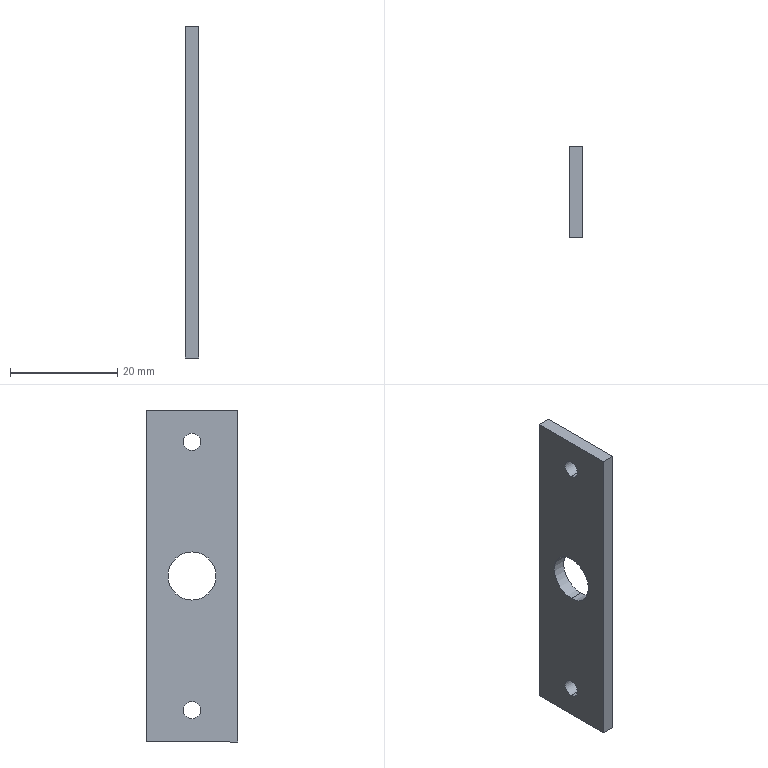Component | SolidWorks | BufferReinforcementPlate(PG50-106)-1 | 1 solid | 12 faces | box 2.5 x 17 x 61.9 mm | volume 2431 mm3 | cylinder 6 | plane 6 | commonest cylinder face diameters 3.2 x4 9 x2
build123d program:
from build123d import *

# Parameters (mm, degrees)
SKETCH1_W           = 61.9
SKETCH1_H           = 17
SKETCH1_R           = 1.6
SKETCH1_R_2         = 4.5
BOSS_EXTRUDE1_DEPTH = 2.5


with BuildPart() as part:
    # Sketch1 → Boss-Extrude1 (new body)
    with BuildSketch(Plane.XY):
        Rectangle(SKETCH1_W, SKETCH1_H)
        with Locations((-25, 0)):
            Circle(SKETCH1_R, mode=Mode.SUBTRACT)
        with Locations((25, 0)):
            Circle(SKETCH1_R, mode=Mode.SUBTRACT)
        Circle(SKETCH1_R_2, mode=Mode.SUBTRACT)
    extrude(amount=BOSS_EXTRUDE1_DEPTH)


solid = part.part

# Placed as in the assembly
solid = solid.moved(Location((919.318, -246.799, -300), (0, 90, 0)))
STEP:
#1=COLOUR_RGB('',0.7922,0.8196,0.9333);
#2=FILL_AREA_STYLE_COLOUR('',#1);
#3=FILL_AREA_STYLE('',(#2));
#4=SURFACE_STYLE_FILL_AREA(#3);
#5=SURFACE_SIDE_STYLE('',(#4));
#6=SURFACE_STYLE_USAGE(.BOTH.,#5);
#7=PRESENTATION_STYLE_ASSIGNMENT((#6));
#8=CARTESIAN_POINT('',(36.194,-9.716,-11.988));
#9=VERTEX_POINT('',#8);
#10=CARTESIAN_POINT('',(36.194,-9.716,-11.634));
#11=VERTEX_POINT('',#10);
#12=CARTESIAN_POINT('',(36.194,-9.716,-11.811));
#13=DIRECTION('',(-1.,0.,-0.));
#14=DIRECTION('',(0.,-0.,1.));
#15=AXIS2_PLACEMENT_3D('',#12,#13,#14);
#16=CIRCLE('',#15,0.1772);
#17=EDGE_CURVE('',#9,#11,#16,.T.);
#18=ORIENTED_EDGE('',*,*,#17,.T.);
#19=CARTESIAN_POINT('',(36.292,-9.716,-11.634));
#20=VERTEX_POINT('',#19);
#21=CARTESIAN_POINT('',(36.194,-9.716,-11.634));
#22=DIRECTION('',(1.,-0.,0.));
#23=VECTOR('',#22,39.37);
#24=LINE('',#21,#23);
#25=EDGE_CURVE('',#11,#20,#24,.T.);
#26=ORIENTED_EDGE('',*,*,#25,.T.);
#27=CARTESIAN_POINT('',(36.292,-9.716,-11.988));
#28=VERTEX_POINT('',#27);
#29=CARTESIAN_POINT('',(36.292,-9.716,-11.811));
#30=DIRECTION('',(-1.,0.,-0.));
#31=DIRECTION('',(0.,-0.,1.));
#32=AXIS2_PLACEMENT_3D('',#29,#30,#31);
#33=CIRCLE('',#32,0.1772);
#34=EDGE_CURVE('',#28,#20,#33,.T.);
#35=ORIENTED_EDGE('',*,*,#34,.F.);
#36=CARTESIAN_POINT('',(36.194,-9.716,-11.988));
#37=DIRECTION('',(1.,-0.,0.));
#38=VECTOR('',#37,39.37);
#39=LINE('',#36,#38);
#40=EDGE_CURVE('',#9,#28,#39,.T.);
#41=ORIENTED_EDGE('',*,*,#40,.F.);
#42=EDGE_LOOP('',(#18,#26,#35,#41));
#43=FACE_OUTER_BOUND('',#42,.T.);
#44=CARTESIAN_POINT('',(36.194,-9.716,-11.811));
#45=DIRECTION('',(1.,-0.,0.));
#46=DIRECTION('',(0.,0.,-1.));
#47=AXIS2_PLACEMENT_3D('',#44,#45,#46);
#48=CYLINDRICAL_SURFACE('',#47,0.1772);
#49=ADVANCED_FACE('',(#43),#48,.F.);
#50=CARTESIAN_POINT('',(36.194,-9.716,-10.89));
#51=VERTEX_POINT('',#50);
#52=CARTESIAN_POINT('',(36.194,-9.716,-10.764));
#53=VERTEX_POINT('',#52);
#54=CARTESIAN_POINT('',(36.194,-9.716,-10.827));
#55=DIRECTION('',(-1.,0.,-0.));
#56=DIRECTION('',(0.,0.,1.));
#57=AXIS2_PLACEMENT_3D('',#54,#55,#56);
#58=CIRCLE('',#57,0.06299);
#59=EDGE_CURVE('',#51,#53,#58,.T.);
#60=ORIENTED_EDGE('',*,*,#59,.T.);
#61=CARTESIAN_POINT('',(36.292,-9.716,-10.764));
#62=VERTEX_POINT('',#61);
#63=CARTESIAN_POINT('',(36.194,-9.716,-10.764));
#64=DIRECTION('',(1.,-0.,0.));
#65=VECTOR('',#64,39.37);
#66=LINE('',#63,#65);
#67=EDGE_CURVE('',#53,#62,#66,.T.);
#68=ORIENTED_EDGE('',*,*,#67,.T.);
#69=CARTESIAN_POINT('',(36.292,-9.716,-10.89));
#70=VERTEX_POINT('',#69);
#71=CARTESIAN_POINT('',(36.292,-9.716,-10.827));
#72=DIRECTION('',(-1.,0.,-0.));
#73=DIRECTION('',(0.,0.,1.));
#74=AXIS2_PLACEMENT_3D('',#71,#72,#73);
#75=CIRCLE('',#74,0.06299);
#76=EDGE_CURVE('',#70,#62,#75,.T.);
#77=ORIENTED_EDGE('',*,*,#76,.F.);
#78=CARTESIAN_POINT('',(36.194,-9.716,-10.89));
#79=DIRECTION('',(1.,-0.,0.));
#80=VECTOR('',#79,39.37);
#81=LINE('',#78,#80);
#82=EDGE_CURVE('',#51,#70,#81,.T.);
#83=ORIENTED_EDGE('',*,*,#82,.F.);
#84=EDGE_LOOP('',(#60,#68,#77,#83));
#85=FACE_OUTER_BOUND('',#84,.T.);
#86=CARTESIAN_POINT('',(36.194,-9.716,-10.827));
#87=DIRECTION('',(1.,-0.,0.));
#88=DIRECTION('',(0.,0.,-1.));
#89=AXIS2_PLACEMENT_3D('',#86,#87,#88);
#90=CYLINDRICAL_SURFACE('',#89,0.06299);
#91=ADVANCED_FACE('',(#85),#90,.F.);
#92=CARTESIAN_POINT('',(36.194,-9.716,-12.858));
#93=VERTEX_POINT('',#92);
#94=CARTESIAN_POINT('',(36.194,-9.716,-12.732));
#95=VERTEX_POINT('',#94);
#96=CARTESIAN_POINT('',(36.194,-9.716,-12.795));
#97=DIRECTION('',(-1.,0.,-0.));
#98=DIRECTION('',(0.,0.,1.));
#99=AXIS2_PLACEMENT_3D('',#96,#97,#98);
#100=CIRCLE('',#99,0.06299);
#101=EDGE_CURVE('',#93,#95,#100,.T.);
#102=ORIENTED_EDGE('',*,*,#101,.T.);
#103=CARTESIAN_POINT('',(36.292,-9.716,-12.732));
#104=VERTEX_POINT('',#103);
#105=CARTESIAN_POINT('',(36.194,-9.716,-12.732));
#106=DIRECTION('',(1.,-0.,0.));
#107=VECTOR('',#106,39.37);
#108=LINE('',#105,#107);
#109=EDGE_CURVE('',#95,#104,#108,.T.);
#110=ORIENTED_EDGE('',*,*,#109,.T.);
#111=CARTESIAN_POINT('',(36.292,-9.716,-12.858));
#112=VERTEX_POINT('',#111);
#113=CARTESIAN_POINT('',(36.292,-9.716,-12.795));
#114=DIRECTION('',(-1.,0.,-0.));
#115=DIRECTION('',(0.,0.,1.));
#116=AXIS2_PLACEMENT_3D('',#113,#114,#115);
#117=CIRCLE('',#116,0.06299);
#118=EDGE_CURVE('',#112,#104,#117,.T.);
#119=ORIENTED_EDGE('',*,*,#118,.F.);
#120=CARTESIAN_POINT('',(36.194,-9.716,-12.858));
#121=DIRECTION('',(1.,-0.,0.));
#122=VECTOR('',#121,39.37);
#123=LINE('',#120,#122);
#124=EDGE_CURVE('',#93,#112,#123,.T.);
#125=ORIENTED_EDGE('',*,*,#124,.F.);
#126=EDGE_LOOP('',(#102,#110,#119,#125));
#127=FACE_OUTER_BOUND('',#126,.T.);
#128=CARTESIAN_POINT('',(36.194,-9.716,-12.795));
#129=DIRECTION('',(1.,-0.,0.));
#130=DIRECTION('',(0.,0.,-1.));
#131=AXIS2_PLACEMENT_3D('',#128,#129,#130);
#132=CYLINDRICAL_SURFACE('',#131,0.06299);
#133=ADVANCED_FACE('',(#127),#132,.F.);
#134=ORIENTED_EDGE('',*,*,#59,.F.);
#135=CARTESIAN_POINT('',(36.194,-9.716,-10.827));
#136=DIRECTION('',(-1.,0.,-0.));
#137=DIRECTION('',(0.,0.,1.));
#138=AXIS2_PLACEMENT_3D('',#135,#136,#137);
#139=CIRCLE('',#138,0.06299);
#140=EDGE_CURVE('',#53,#51,#139,.T.);
#141=ORIENTED_EDGE('',*,*,#140,.F.);
#142=EDGE_LOOP('',(#134,#141));
#143=FACE_BOUND('',#142,.T.);
#144=CARTESIAN_POINT('',(36.194,-9.382,-13.03));
#145=VERTEX_POINT('',#144);
#146=CARTESIAN_POINT('',(36.194,-10.051,-13.03));
#147=VERTEX_POINT('',#146);
#148=CARTESIAN_POINT('',(36.194,-10.051,-13.03));
#149=DIRECTION('',(-0.,-1.,-0.));
#150=VECTOR('',#149,39.37);
#151=LINE('',#148,#150);
#152=EDGE_CURVE('',#145,#147,#151,.T.);
#153=ORIENTED_EDGE('',*,*,#152,.T.);
#154=CARTESIAN_POINT('',(36.194,-10.051,-10.593));
#155=VERTEX_POINT('',#154);
#156=CARTESIAN_POINT('',(36.194,-10.051,-10.593));
#157=DIRECTION('',(-0.,-0.,1.));
#158=VECTOR('',#157,39.37);
#159=LINE('',#156,#158);
#160=EDGE_CURVE('',#147,#155,#159,.T.);
#161=ORIENTED_EDGE('',*,*,#160,.T.);
#162=CARTESIAN_POINT('',(36.194,-9.382,-10.593));
#163=VERTEX_POINT('',#162);
#164=CARTESIAN_POINT('',(36.194,-9.382,-10.593));
#165=DIRECTION('',(0.,1.,0.));
#166=VECTOR('',#165,39.37);
#167=LINE('',#164,#166);
#168=EDGE_CURVE('',#155,#163,#167,.T.);
#169=ORIENTED_EDGE('',*,*,#168,.T.);
#170=CARTESIAN_POINT('',(36.194,-9.382,-13.03));
#171=DIRECTION('',(0.,0.,-1.));
#172=VECTOR('',#171,39.37);
#173=LINE('',#170,#172);
#174=EDGE_CURVE('',#163,#145,#173,.T.);
#175=ORIENTED_EDGE('',*,*,#174,.T.);
#176=EDGE_LOOP('',(#153,#161,#169,#175));
#177=FACE_OUTER_BOUND('',#176,.T.);
#178=ORIENTED_EDGE('',*,*,#101,.F.);
#179=CARTESIAN_POINT('',(36.194,-9.716,-12.795));
#180=DIRECTION('',(-1.,0.,-0.));
#181=DIRECTION('',(0.,0.,1.));
#182=AXIS2_PLACEMENT_3D('',#179,#180,#181);
#183=CIRCLE('',#182,0.06299);
#184=EDGE_CURVE('',#95,#93,#183,.T.);
#185=ORIENTED_EDGE('',*,*,#184,.F.);
#186=EDGE_LOOP('',(#178,#185));
#187=FACE_BOUND('',#186,.T.);
#188=ORIENTED_EDGE('',*,*,#17,.F.);
#189=CARTESIAN_POINT('',(36.194,-9.716,-11.811));
#190=DIRECTION('',(-1.,0.,-0.));
#191=DIRECTION('',(0.,-0.,1.));
#192=AXIS2_PLACEMENT_3D('',#189,#190,#191);
#193=CIRCLE('',#192,0.1772);
#194=EDGE_CURVE('',#11,#9,#193,.T.);
#195=ORIENTED_EDGE('',*,*,#194,.F.);
#196=EDGE_LOOP('',(#188,#195));
#197=FACE_BOUND('',#196,.T.);
#198=CARTESIAN_POINT('',(36.194,-9.716,-11.811));
#199=DIRECTION('',(1.,-0.,0.));
#200=DIRECTION('',(0.,0.,-1.));
#201=AXIS2_PLACEMENT_3D('',#198,#199,#200);
#202=PLANE('',#201);
#203=ADVANCED_FACE('',(#143,#177,#187,#197),#202,.F.);
#204=ORIENTED_EDGE('',*,*,#76,.T.);
#205=CARTESIAN_POINT('',(36.292,-9.716,-10.827));
#206=DIRECTION('',(-1.,0.,-0.));
#207=DIRECTION('',(0.,0.,1.));
#208=AXIS2_PLACEMENT_3D('',#205,#206,#207);
#209=CIRCLE('',#208,0.06299);
#210=EDGE_CURVE('',#62,#70,#209,.T.);
#211=ORIENTED_EDGE('',*,*,#210,.T.);
#212=EDGE_LOOP('',(#204,#211));
#213=FACE_BOUND('',#212,.T.);
#214=CARTESIAN_POINT('',(36.292,-9.382,-13.03));
#215=VERTEX_POINT('',#214);
#216=CARTESIAN_POINT('',(36.292,-10.051,-13.03));
#217=VERTEX_POINT('',#216);
#218=CARTESIAN_POINT('',(36.292,-10.051,-13.03));
#219=DIRECTION('',(-0.,-1.,-0.));
#220=VECTOR('',#219,39.37);
#221=LINE('',#218,#220);
#222=EDGE_CURVE('',#215,#217,#221,.T.);
#223=ORIENTED_EDGE('',*,*,#222,.F.);
#224=CARTESIAN_POINT('',(36.292,-9.382,-10.593));
#225=VERTEX_POINT('',#224);
#226=CARTESIAN_POINT('',(36.292,-9.382,-13.03));
#227=DIRECTION('',(0.,0.,-1.));
#228=VECTOR('',#227,39.37);
#229=LINE('',#226,#228);
#230=EDGE_CURVE('',#225,#215,#229,.T.);
#231=ORIENTED_EDGE('',*,*,#230,.F.);
#232=CARTESIAN_POINT('',(36.292,-10.051,-10.593));
#233=VERTEX_POINT('',#232);
#234=CARTESIAN_POINT('',(36.292,-9.382,-10.593));
#235=DIRECTION('',(0.,1.,0.));
#236=VECTOR('',#235,39.37);
#237=LINE('',#234,#236);
#238=EDGE_CURVE('',#233,#225,#237,.T.);
#239=ORIENTED_EDGE('',*,*,#238,.F.);
#240=CARTESIAN_POINT('',(36.292,-10.051,-10.593));
#241=DIRECTION('',(-0.,-0.,1.));
#242=VECTOR('',#241,39.37);
#243=LINE('',#240,#242);
#244=EDGE_CURVE('',#217,#233,#243,.T.);
#245=ORIENTED_EDGE('',*,*,#244,.F.);
#246=EDGE_LOOP('',(#223,#231,#239,#245));
#247=FACE_OUTER_BOUND('',#246,.T.);
#248=ORIENTED_EDGE('',*,*,#118,.T.);
#249=CARTESIAN_POINT('',(36.292,-9.716,-12.795));
#250=DIRECTION('',(-1.,0.,-0.));
#251=DIRECTION('',(0.,0.,1.));
#252=AXIS2_PLACEMENT_3D('',#249,#250,#251);
#253=CIRCLE('',#252,0.06299);
#254=EDGE_CURVE('',#104,#112,#253,.T.);
#255=ORIENTED_EDGE('',*,*,#254,.T.);
#256=EDGE_LOOP('',(#248,#255));
#257=FACE_BOUND('',#256,.T.);
#258=ORIENTED_EDGE('',*,*,#34,.T.);
#259=CARTESIAN_POINT('',(36.292,-9.716,-11.811));
#260=DIRECTION('',(-1.,0.,-0.));
#261=DIRECTION('',(0.,-0.,1.));
#262=AXIS2_PLACEMENT_3D('',#259,#260,#261);
#263=CIRCLE('',#262,0.1772);
#264=EDGE_CURVE('',#20,#28,#263,.T.);
#265=ORIENTED_EDGE('',*,*,#264,.T.);
#266=EDGE_LOOP('',(#258,#265));
#267=FACE_BOUND('',#266,.T.);
#268=CARTESIAN_POINT('',(36.292,-9.716,-11.811));
#269=DIRECTION('',(1.,-0.,0.));
#270=DIRECTION('',(0.,0.,-1.));
#271=AXIS2_PLACEMENT_3D('',#268,#269,#270);
#272=PLANE('',#271);
#273=ADVANCED_FACE('',(#213,#247,#257,#267),#272,.T.);
#274=ORIENTED_EDGE('',*,*,#222,.T.);
#275=CARTESIAN_POINT('',(36.194,-10.051,-13.03));
#276=DIRECTION('',(1.,-0.,0.));
#277=VECTOR('',#276,39.37);
#278=LINE('',#275,#277);
#279=EDGE_CURVE('',#147,#217,#278,.T.);
#280=ORIENTED_EDGE('',*,*,#279,.F.);
#281=ORIENTED_EDGE('',*,*,#152,.F.);
#282=CARTESIAN_POINT('',(36.194,-9.382,-13.03));
#283=DIRECTION('',(1.,-0.,0.));
#284=VECTOR('',#283,39.37);
#285=LINE('',#282,#284);
#286=EDGE_CURVE('',#145,#215,#285,.T.);
#287=ORIENTED_EDGE('',*,*,#286,.T.);
#288=EDGE_LOOP('',(#274,#280,#281,#287));
#289=FACE_OUTER_BOUND('',#288,.T.);
#290=CARTESIAN_POINT('',(36.194,-10.051,-13.03));
#291=DIRECTION('',(-0.,-0.,1.));
#292=DIRECTION('',(1.,-0.,0.));
#293=AXIS2_PLACEMENT_3D('',#290,#291,#292);
#294=PLANE('',#293);
#295=ADVANCED_FACE('',(#289),#294,.F.);
#296=ORIENTED_EDGE('',*,*,#244,.T.);
#297=CARTESIAN_POINT('',(36.194,-10.051,-10.593));
#298=DIRECTION('',(1.,-0.,0.));
#299=VECTOR('',#298,39.37);
#300=LINE('',#297,#299);
#301=EDGE_CURVE('',#155,#233,#300,.T.);
#302=ORIENTED_EDGE('',*,*,#301,.F.);
#303=ORIENTED_EDGE('',*,*,#160,.F.);
#304=ORIENTED_EDGE('',*,*,#279,.T.);
#305=EDGE_LOOP('',(#296,#302,#303,#304));
#306=FACE_OUTER_BOUND('',#305,.T.);
#307=CARTESIAN_POINT('',(36.194,-10.051,-10.593));
#308=DIRECTION('',(0.,1.,0.));
#309=DIRECTION('',(-1.,0.,-0.));
#310=AXIS2_PLACEMENT_3D('',#307,#308,#309);
#311=PLANE('',#310);
#312=ADVANCED_FACE('',(#306),#311,.F.);
#313=ORIENTED_EDGE('',*,*,#238,.T.);
#314=CARTESIAN_POINT('',(36.194,-9.382,-10.593));
#315=DIRECTION('',(1.,-0.,0.));
#316=VECTOR('',#315,39.37);
#317=LINE('',#314,#316);
#318=EDGE_CURVE('',#163,#225,#317,.T.);
#319=ORIENTED_EDGE('',*,*,#318,.F.);
#320=ORIENTED_EDGE('',*,*,#168,.F.);
#321=ORIENTED_EDGE('',*,*,#301,.T.);
#322=EDGE_LOOP('',(#313,#319,#320,#321));
#323=FACE_OUTER_BOUND('',#322,.T.);
#324=CARTESIAN_POINT('',(36.194,-9.382,-10.593));
#325=DIRECTION('',(0.,0.,-1.));
#326=DIRECTION('',(-1.,0.,-0.));
#327=AXIS2_PLACEMENT_3D('',#324,#325,#326);
#328=PLANE('',#327);
#329=ADVANCED_FACE('',(#323),#328,.F.);
#330=ORIENTED_EDGE('',*,*,#230,.T.);
#331=ORIENTED_EDGE('',*,*,#286,.F.);
#332=ORIENTED_EDGE('',*,*,#174,.F.);
#333=ORIENTED_EDGE('',*,*,#318,.T.);
#334=EDGE_LOOP('',(#330,#331,#332,#333));
#335=FACE_OUTER_BOUND('',#334,.T.);
#336=CARTESIAN_POINT('',(36.194,-9.382,-13.03));
#337=DIRECTION('',(-0.,-1.,-0.));
#338=DIRECTION('',(1.,-0.,0.));
#339=AXIS2_PLACEMENT_3D('',#336,#337,#338);
#340=PLANE('',#339);
#341=ADVANCED_FACE('',(#335),#340,.F.);
#342=ORIENTED_EDGE('',*,*,#109,.F.);
#343=ORIENTED_EDGE('',*,*,#184,.T.);
#344=ORIENTED_EDGE('',*,*,#124,.T.);
#345=ORIENTED_EDGE('',*,*,#254,.F.);
#346=EDGE_LOOP('',(#342,#343,#344,#345));
#347=FACE_OUTER_BOUND('',#346,.T.);
#348=CARTESIAN_POINT('',(36.194,-9.716,-12.795));
#349=DIRECTION('',(1.,-0.,0.));
#350=DIRECTION('',(0.,0.,-1.));
#351=AXIS2_PLACEMENT_3D('',#348,#349,#350);
#352=CYLINDRICAL_SURFACE('',#351,0.06299);
#353=ADVANCED_FACE('',(#347),#352,.F.);
#354=ORIENTED_EDGE('',*,*,#67,.F.);
#355=ORIENTED_EDGE('',*,*,#140,.T.);
#356=ORIENTED_EDGE('',*,*,#82,.T.);
#357=ORIENTED_EDGE('',*,*,#210,.F.);
#358=EDGE_LOOP('',(#354,#355,#356,#357));
#359=FACE_OUTER_BOUND('',#358,.T.);
#360=CARTESIAN_POINT('',(36.194,-9.716,-10.827));
#361=DIRECTION('',(1.,-0.,0.));
#362=DIRECTION('',(0.,0.,-1.));
#363=AXIS2_PLACEMENT_3D('',#360,#361,#362);
#364=CYLINDRICAL_SURFACE('',#363,0.06299);
#365=ADVANCED_FACE('',(#359),#364,.F.);
#366=ORIENTED_EDGE('',*,*,#25,.F.);
#367=ORIENTED_EDGE('',*,*,#194,.T.);
#368=ORIENTED_EDGE('',*,*,#40,.T.);
#369=ORIENTED_EDGE('',*,*,#264,.F.);
#370=EDGE_LOOP('',(#366,#367,#368,#369));
#371=FACE_OUTER_BOUND('',#370,.T.);
#372=CARTESIAN_POINT('',(36.194,-9.716,-11.811));
#373=DIRECTION('',(1.,-0.,0.));
#374=DIRECTION('',(0.,0.,-1.));
#375=AXIS2_PLACEMENT_3D('',#372,#373,#374);
#376=CYLINDRICAL_SURFACE('',#375,0.1772);
#377=ADVANCED_FACE('',(#371),#376,.F.);
#378=CLOSED_SHELL('',(#49,#91,#133,#203,#273,#295,#312,#329,#341,#353,#365,#377));
#379=MANIFOLD_SOLID_BREP('',#378);
#380=STYLED_ITEM('',(#7),#379);
#381=(LENGTH_UNIT()NAMED_UNIT(*)SI_UNIT($,.METRE.));
#382=LENGTH_MEASURE_WITH_UNIT(LENGTH_MEASURE(0.0254),#381);
#383=DIMENSIONAL_EXPONENTS(1.,0.,0.,0.,0.,0.,0.);
#384=(CONVERSION_BASED_UNIT('',#382)LENGTH_UNIT()NAMED_UNIT(#383));
#385=UNCERTAINTY_MEASURE_WITH_UNIT(LENGTH_MEASURE(0.00001),#384,'','');
#386=(NAMED_UNIT(*)PLANE_ANGLE_UNIT()SI_UNIT($,.RADIAN.));
#387=(NAMED_UNIT(*)SI_UNIT($,.STERADIAN.)SOLID_ANGLE_UNIT());
#388=(GEOMETRIC_REPRESENTATION_CONTEXT(3)GLOBAL_UNCERTAINTY_ASSIGNED_CONTEXT((#385))GLOBAL_UNIT_ASSIGNED_CONTEXT((#384,#386,#387))REPRESENTATION_CONTEXT('',''));
#389=MECHANICAL_DESIGN_GEOMETRIC_PRESENTATION_REPRESENTATION('',(#380),#388);
#390=CARTESIAN_POINT('',(0.,0.,0.));
#391=DIRECTION('',(0.,0.,1.));
#392=DIRECTION('',(1.,0.,0.));
#393=AXIS2_PLACEMENT_3D('',#390,#391,#392);
#394=(LENGTH_UNIT()NAMED_UNIT(*)SI_UNIT($,.METRE.));
#395=LENGTH_MEASURE_WITH_UNIT(LENGTH_MEASURE(0.0254),#394);
#396=DIMENSIONAL_EXPONENTS(1.,0.,0.,0.,0.,0.,0.);
#397=(CONVERSION_BASED_UNIT('',#395)LENGTH_UNIT()NAMED_UNIT(#396));
#398=UNCERTAINTY_MEASURE_WITH_UNIT(LENGTH_MEASURE(0.00001),#397,'','');
#399=(NAMED_UNIT(*)PLANE_ANGLE_UNIT()SI_UNIT($,.RADIAN.));
#400=(NAMED_UNIT(*)SI_UNIT($,.STERADIAN.)SOLID_ANGLE_UNIT());
#401=(GEOMETRIC_REPRESENTATION_CONTEXT(3)GLOBAL_UNCERTAINTY_ASSIGNED_CONTEXT((#398))GLOBAL_UNIT_ASSIGNED_CONTEXT((#397,#399,#400))REPRESENTATION_CONTEXT('',''));
#402=ADVANCED_BREP_SHAPE_REPRESENTATION('',(#379,#393),#401);
#403=PRESENTATION_LAYER_ASSIGNMENT('','',(#380));